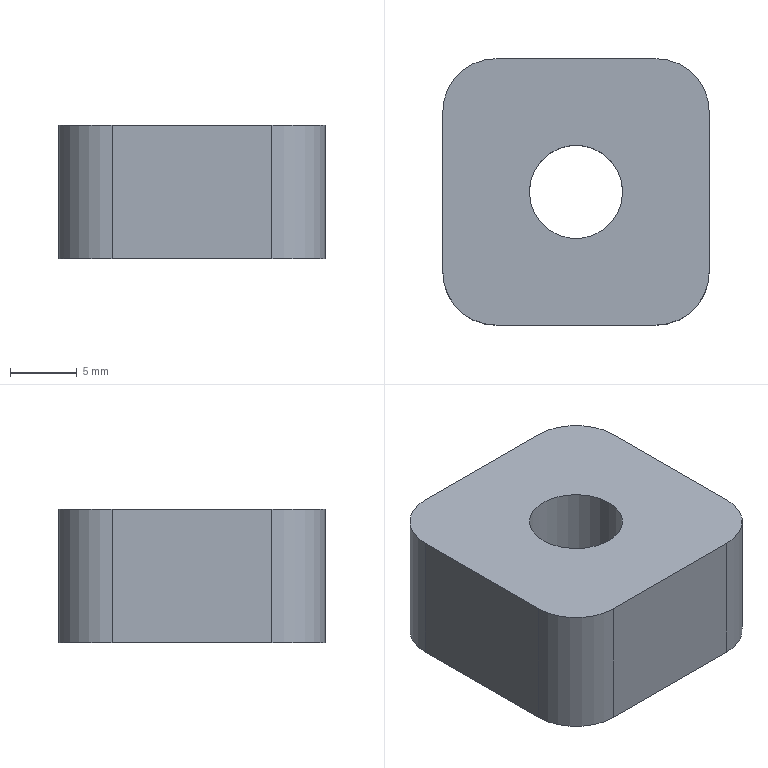Component | NX | FIX_BLOCK_3 | 1 solid | 11 faces | box 20 x 20 x 10 mm | volume 3478 mm3 | plane 6 | cylinder 5 | commonest cylinder face diameters 8 x4 7 x1
STEP:
#1=CARTESIAN_POINT('',(0.,0.,0.));
#2=DIRECTION('',(0.,0.,1.));
#3=DIRECTION('',(1.,0.,0.));
#4=AXIS2_PLACEMENT_3D('',#1,#2,#3);
#5=CARTESIAN_POINT('',(-10.,106.,0.));
#6=VERTEX_POINT('',#5);
#7=CARTESIAN_POINT('',(-10.,94.,0.));
#8=VERTEX_POINT('',#7);
#9=CARTESIAN_POINT('',(-10.,110.,0.));
#10=DIRECTION('',(0.,-1.,0.));
#11=VECTOR('',#10,1.);
#12=LINE('',#9,#11);
#13=CARTESIAN_POINT('',(-10.,110.,10.));
#14=DIRECTION('',(1.,0.,0.));
#15=DIRECTION('',(0.,0.,-1.));
#16=AXIS2_PLACEMENT_3D('',#13,#14,#15);
#17=PLANE('',#16);
#18=CARTESIAN_POINT('',(10.,0.));
#19=DIRECTION('',(0.,-1.));
#20=VECTOR('',#19,1.);
#21=LINE('',#18,#20);
#22=(GEOMETRIC_REPRESENTATION_CONTEXT(2)PARAMETRIC_REPRESENTATION_CONTEXT()REPRESENTATION_CONTEXT('',''));
#23=DEFINITIONAL_REPRESENTATION('',(#21),#22);
#24=PCURVE('',#17,#23);
#25=CARTESIAN_POINT('',(0.,100.,0.));
#26=DIRECTION('',(0.,0.,1.));
#27=DIRECTION('',(1.,0.,0.));
#28=AXIS2_PLACEMENT_3D('',#25,#26,#27);
#29=PLANE('',#28);
#30=CARTESIAN_POINT('',(-10.,10.));
#31=DIRECTION('',(0.,-1.));
#32=VECTOR('',#31,1.);
#33=LINE('',#30,#32);
#34=(GEOMETRIC_REPRESENTATION_CONTEXT(2)PARAMETRIC_REPRESENTATION_CONTEXT()REPRESENTATION_CONTEXT('',''));
#35=DEFINITIONAL_REPRESENTATION('',(#33),#34);
#36=PCURVE('',#29,#35);
#37=SURFACE_CURVE('',#12,(#24,#36),.PCURVE_S1.);
#38=EDGE_CURVE('',#6,#8,#37,.T.);
#39=ORIENTED_EDGE('',*,*,#38,.T.);
#40=CARTESIAN_POINT('',(-10.,94.,10.));
#41=VERTEX_POINT('',#40);
#42=CARTESIAN_POINT('',(-10.,94.,10.));
#43=DIRECTION('',(0.,0.,1.));
#44=VECTOR('',#43,1.);
#45=LINE('',#42,#44);
#46=CARTESIAN_POINT('',(0.,-16.));
#47=DIRECTION('',(-1.,0.));
#48=VECTOR('',#47,1.);
#49=LINE('',#46,#48);
#50=(GEOMETRIC_REPRESENTATION_CONTEXT(2)PARAMETRIC_REPRESENTATION_CONTEXT()REPRESENTATION_CONTEXT('',''));
#51=DEFINITIONAL_REPRESENTATION('',(#49),#50);
#52=PCURVE('',#17,#51);
#53=CARTESIAN_POINT('',(-6.,94.,10.));
#54=DIRECTION('',(0.,0.,-1.));
#55=DIRECTION('',(-1.,0.,0.));
#56=AXIS2_PLACEMENT_3D('',#53,#54,#55);
#57=CYLINDRICAL_SURFACE('',#56,4.);
#58=CARTESIAN_POINT('',(6.283,0.));
#59=DIRECTION('',(0.,-1.));
#60=VECTOR('',#59,1.);
#61=LINE('',#58,#60);
#62=(GEOMETRIC_REPRESENTATION_CONTEXT(2)PARAMETRIC_REPRESENTATION_CONTEXT()REPRESENTATION_CONTEXT('',''));
#63=DEFINITIONAL_REPRESENTATION('',(#61),#62);
#64=PCURVE('',#57,#63);
#65=SURFACE_CURVE('',#45,(#52,#64),.PCURVE_S1.);
#66=EDGE_CURVE('',#8,#41,#65,.T.);
#67=ORIENTED_EDGE('',*,*,#66,.T.);
#68=CARTESIAN_POINT('',(-10.,106.,10.));
#69=VERTEX_POINT('',#68);
#70=CARTESIAN_POINT('',(-10.,110.,10.));
#71=DIRECTION('',(0.,-1.,0.));
#72=VECTOR('',#71,1.);
#73=LINE('',#70,#72);
#74=CARTESIAN_POINT('',(0.,0.));
#75=DIRECTION('',(0.,-1.));
#76=VECTOR('',#75,1.);
#77=LINE('',#74,#76);
#78=(GEOMETRIC_REPRESENTATION_CONTEXT(2)PARAMETRIC_REPRESENTATION_CONTEXT()REPRESENTATION_CONTEXT('',''));
#79=DEFINITIONAL_REPRESENTATION('',(#77),#78);
#80=PCURVE('',#17,#79);
#81=CARTESIAN_POINT('',(0.,100.,10.));
#82=DIRECTION('',(0.,0.,1.));
#83=DIRECTION('',(1.,0.,0.));
#84=AXIS2_PLACEMENT_3D('',#81,#82,#83);
#85=PLANE('',#84);
#86=CARTESIAN_POINT('',(-10.,10.));
#87=DIRECTION('',(0.,-1.));
#88=VECTOR('',#87,1.);
#89=LINE('',#86,#88);
#90=(GEOMETRIC_REPRESENTATION_CONTEXT(2)PARAMETRIC_REPRESENTATION_CONTEXT()REPRESENTATION_CONTEXT('',''));
#91=DEFINITIONAL_REPRESENTATION('',(#89),#90);
#92=PCURVE('',#85,#91);
#93=SURFACE_CURVE('',#73,(#80,#92),.PCURVE_S1.);
#94=EDGE_CURVE('',#69,#41,#93,.T.);
#95=ORIENTED_EDGE('',*,*,#94,.F.);
#96=CARTESIAN_POINT('',(-10.,106.,10.));
#97=DIRECTION('',(0.,0.,-1.));
#98=VECTOR('',#97,1.);
#99=LINE('',#96,#98);
#100=CARTESIAN_POINT('',(0.,-4.));
#101=DIRECTION('',(1.,0.));
#102=VECTOR('',#101,1.);
#103=LINE('',#100,#102);
#104=(GEOMETRIC_REPRESENTATION_CONTEXT(2)PARAMETRIC_REPRESENTATION_CONTEXT()REPRESENTATION_CONTEXT('',''));
#105=DEFINITIONAL_REPRESENTATION('',(#103),#104);
#106=PCURVE('',#17,#105);
#107=CARTESIAN_POINT('',(-6.,106.,10.));
#108=DIRECTION('',(0.,0.,-1.));
#109=DIRECTION('',(-1.,0.,0.));
#110=AXIS2_PLACEMENT_3D('',#107,#108,#109);
#111=CYLINDRICAL_SURFACE('',#110,4.);
#112=CARTESIAN_POINT('',(0.,0.));
#113=DIRECTION('',(0.,1.));
#114=VECTOR('',#113,1.);
#115=LINE('',#112,#114);
#116=(GEOMETRIC_REPRESENTATION_CONTEXT(2)PARAMETRIC_REPRESENTATION_CONTEXT()REPRESENTATION_CONTEXT('',''));
#117=DEFINITIONAL_REPRESENTATION('',(#115),#116);
#118=PCURVE('',#111,#117);
#119=SURFACE_CURVE('',#99,(#106,#118),.PCURVE_S1.);
#120=EDGE_CURVE('',#69,#6,#119,.T.);
#121=ORIENTED_EDGE('',*,*,#120,.T.);
#122=EDGE_LOOP('',(#39,#67,#95,#121));
#123=FACE_BOUND('',#122,.T.);
#124=ADVANCED_FACE('',(#123),#17,.F.);
#125=CARTESIAN_POINT('',(-6.,90.,0.));
#126=VERTEX_POINT('',#125);
#127=CARTESIAN_POINT('',(6.,90.,0.));
#128=VERTEX_POINT('',#127);
#129=CARTESIAN_POINT('',(-10.,90.,0.));
#130=DIRECTION('',(1.,0.,0.));
#131=VECTOR('',#130,1.);
#132=LINE('',#129,#131);
#133=CARTESIAN_POINT('',(-10.,90.,10.));
#134=DIRECTION('',(0.,1.,0.));
#135=DIRECTION('',(0.,0.,1.));
#136=AXIS2_PLACEMENT_3D('',#133,#134,#135);
#137=PLANE('',#136);
#138=CARTESIAN_POINT('',(-10.,0.));
#139=DIRECTION('',(0.,1.));
#140=VECTOR('',#139,1.);
#141=LINE('',#138,#140);
#142=(GEOMETRIC_REPRESENTATION_CONTEXT(2)PARAMETRIC_REPRESENTATION_CONTEXT()REPRESENTATION_CONTEXT('',''));
#143=DEFINITIONAL_REPRESENTATION('',(#141),#142);
#144=PCURVE('',#137,#143);
#145=CARTESIAN_POINT('',(-10.,-10.));
#146=DIRECTION('',(1.,0.));
#147=VECTOR('',#146,1.);
#148=LINE('',#145,#147);
#149=(GEOMETRIC_REPRESENTATION_CONTEXT(2)PARAMETRIC_REPRESENTATION_CONTEXT()REPRESENTATION_CONTEXT('',''));
#150=DEFINITIONAL_REPRESENTATION('',(#148),#149);
#151=PCURVE('',#29,#150);
#152=SURFACE_CURVE('',#132,(#144,#151),.PCURVE_S1.);
#153=EDGE_CURVE('',#126,#128,#152,.T.);
#154=ORIENTED_EDGE('',*,*,#153,.T.);
#155=CARTESIAN_POINT('',(6.,90.,10.));
#156=VERTEX_POINT('',#155);
#157=CARTESIAN_POINT('',(6.,90.,10.));
#158=DIRECTION('',(0.,0.,1.));
#159=VECTOR('',#158,1.);
#160=LINE('',#157,#159);
#161=CARTESIAN_POINT('',(0.,16.));
#162=DIRECTION('',(1.,0.));
#163=VECTOR('',#162,1.);
#164=LINE('',#161,#163);
#165=(GEOMETRIC_REPRESENTATION_CONTEXT(2)PARAMETRIC_REPRESENTATION_CONTEXT()REPRESENTATION_CONTEXT('',''));
#166=DEFINITIONAL_REPRESENTATION('',(#164),#165);
#167=PCURVE('',#137,#166);
#168=CARTESIAN_POINT('',(6.,94.,10.));
#169=DIRECTION('',(0.,0.,-1.));
#170=DIRECTION('',(-1.,0.,0.));
#171=AXIS2_PLACEMENT_3D('',#168,#169,#170);
#172=CYLINDRICAL_SURFACE('',#171,4.);
#173=CARTESIAN_POINT('',(4.712,0.));
#174=DIRECTION('',(0.,-1.));
#175=VECTOR('',#174,1.);
#176=LINE('',#173,#175);
#177=(GEOMETRIC_REPRESENTATION_CONTEXT(2)PARAMETRIC_REPRESENTATION_CONTEXT()REPRESENTATION_CONTEXT('',''));
#178=DEFINITIONAL_REPRESENTATION('',(#176),#177);
#179=PCURVE('',#172,#178);
#180=SURFACE_CURVE('',#160,(#167,#179),.PCURVE_S1.);
#181=EDGE_CURVE('',#128,#156,#180,.T.);
#182=ORIENTED_EDGE('',*,*,#181,.T.);
#183=CARTESIAN_POINT('',(-6.,90.,10.));
#184=VERTEX_POINT('',#183);
#185=CARTESIAN_POINT('',(-10.,90.,10.));
#186=DIRECTION('',(1.,0.,0.));
#187=VECTOR('',#186,1.);
#188=LINE('',#185,#187);
#189=CARTESIAN_POINT('',(0.,0.));
#190=DIRECTION('',(0.,1.));
#191=VECTOR('',#190,1.);
#192=LINE('',#189,#191);
#193=(GEOMETRIC_REPRESENTATION_CONTEXT(2)PARAMETRIC_REPRESENTATION_CONTEXT()REPRESENTATION_CONTEXT('',''));
#194=DEFINITIONAL_REPRESENTATION('',(#192),#193);
#195=PCURVE('',#137,#194);
#196=CARTESIAN_POINT('',(-10.,-10.));
#197=DIRECTION('',(1.,0.));
#198=VECTOR('',#197,1.);
#199=LINE('',#196,#198);
#200=(GEOMETRIC_REPRESENTATION_CONTEXT(2)PARAMETRIC_REPRESENTATION_CONTEXT()REPRESENTATION_CONTEXT('',''));
#201=DEFINITIONAL_REPRESENTATION('',(#199),#200);
#202=PCURVE('',#85,#201);
#203=SURFACE_CURVE('',#188,(#195,#202),.PCURVE_S1.);
#204=EDGE_CURVE('',#184,#156,#203,.T.);
#205=ORIENTED_EDGE('',*,*,#204,.F.);
#206=CARTESIAN_POINT('',(-6.,90.,10.));
#207=DIRECTION('',(0.,0.,-1.));
#208=VECTOR('',#207,1.);
#209=LINE('',#206,#208);
#210=CARTESIAN_POINT('',(0.,4.));
#211=DIRECTION('',(-1.,0.));
#212=VECTOR('',#211,1.);
#213=LINE('',#210,#212);
#214=(GEOMETRIC_REPRESENTATION_CONTEXT(2)PARAMETRIC_REPRESENTATION_CONTEXT()REPRESENTATION_CONTEXT('',''));
#215=DEFINITIONAL_REPRESENTATION('',(#213),#214);
#216=PCURVE('',#137,#215);
#217=CARTESIAN_POINT('',(4.712,0.));
#218=DIRECTION('',(0.,1.));
#219=VECTOR('',#218,1.);
#220=LINE('',#217,#219);
#221=(GEOMETRIC_REPRESENTATION_CONTEXT(2)PARAMETRIC_REPRESENTATION_CONTEXT()REPRESENTATION_CONTEXT('',''));
#222=DEFINITIONAL_REPRESENTATION('',(#220),#221);
#223=PCURVE('',#57,#222);
#224=SURFACE_CURVE('',#209,(#216,#223),.PCURVE_S1.);
#225=EDGE_CURVE('',#184,#126,#224,.T.);
#226=ORIENTED_EDGE('',*,*,#225,.T.);
#227=EDGE_LOOP('',(#154,#182,#205,#226));
#228=FACE_BOUND('',#227,.T.);
#229=ADVANCED_FACE('',(#228),#137,.F.);
#230=CARTESIAN_POINT('',(10.,94.,10.));
#231=VERTEX_POINT('',#230);
#232=CARTESIAN_POINT('',(10.,106.,10.));
#233=VERTEX_POINT('',#232);
#234=CARTESIAN_POINT('',(10.,90.,10.));
#235=DIRECTION('',(0.,1.,0.));
#236=VECTOR('',#235,1.);
#237=LINE('',#234,#236);
#238=CARTESIAN_POINT('',(10.,90.,10.));
#239=DIRECTION('',(-1.,0.,0.));
#240=DIRECTION('',(0.,0.,1.));
#241=AXIS2_PLACEMENT_3D('',#238,#239,#240);
#242=PLANE('',#241);
#243=CARTESIAN_POINT('',(0.,0.));
#244=DIRECTION('',(0.,1.));
#245=VECTOR('',#244,1.);
#246=LINE('',#243,#245);
#247=(GEOMETRIC_REPRESENTATION_CONTEXT(2)PARAMETRIC_REPRESENTATION_CONTEXT()REPRESENTATION_CONTEXT('',''));
#248=DEFINITIONAL_REPRESENTATION('',(#246),#247);
#249=PCURVE('',#242,#248);
#250=CARTESIAN_POINT('',(10.,-10.));
#251=DIRECTION('',(0.,1.));
#252=VECTOR('',#251,1.);
#253=LINE('',#250,#252);
#254=(GEOMETRIC_REPRESENTATION_CONTEXT(2)PARAMETRIC_REPRESENTATION_CONTEXT()REPRESENTATION_CONTEXT('',''));
#255=DEFINITIONAL_REPRESENTATION('',(#253),#254);
#256=PCURVE('',#85,#255);
#257=SURFACE_CURVE('',#237,(#249,#256),.PCURVE_S1.);
#258=EDGE_CURVE('',#231,#233,#257,.T.);
#259=ORIENTED_EDGE('',*,*,#258,.F.);
#260=CARTESIAN_POINT('',(10.,94.,0.));
#261=VERTEX_POINT('',#260);
#262=CARTESIAN_POINT('',(10.,94.,10.));
#263=DIRECTION('',(0.,0.,-1.));
#264=VECTOR('',#263,1.);
#265=LINE('',#262,#264);
#266=CARTESIAN_POINT('',(0.,4.));
#267=DIRECTION('',(-1.,0.));
#268=VECTOR('',#267,1.);
#269=LINE('',#266,#268);
#270=(GEOMETRIC_REPRESENTATION_CONTEXT(2)PARAMETRIC_REPRESENTATION_CONTEXT()REPRESENTATION_CONTEXT('',''));
#271=DEFINITIONAL_REPRESENTATION('',(#269),#270);
#272=PCURVE('',#242,#271);
#273=CARTESIAN_POINT('',(3.142,0.));
#274=DIRECTION('',(0.,1.));
#275=VECTOR('',#274,1.);
#276=LINE('',#273,#275);
#277=(GEOMETRIC_REPRESENTATION_CONTEXT(2)PARAMETRIC_REPRESENTATION_CONTEXT()REPRESENTATION_CONTEXT('',''));
#278=DEFINITIONAL_REPRESENTATION('',(#276),#277);
#279=PCURVE('',#172,#278);
#280=SURFACE_CURVE('',#265,(#272,#279),.PCURVE_S1.);
#281=EDGE_CURVE('',#231,#261,#280,.T.);
#282=ORIENTED_EDGE('',*,*,#281,.T.);
#283=CARTESIAN_POINT('',(10.,106.,0.));
#284=VERTEX_POINT('',#283);
#285=CARTESIAN_POINT('',(10.,90.,0.));
#286=DIRECTION('',(0.,1.,0.));
#287=VECTOR('',#286,1.);
#288=LINE('',#285,#287);
#289=CARTESIAN_POINT('',(-10.,0.));
#290=DIRECTION('',(0.,1.));
#291=VECTOR('',#290,1.);
#292=LINE('',#289,#291);
#293=(GEOMETRIC_REPRESENTATION_CONTEXT(2)PARAMETRIC_REPRESENTATION_CONTEXT()REPRESENTATION_CONTEXT('',''));
#294=DEFINITIONAL_REPRESENTATION('',(#292),#293);
#295=PCURVE('',#242,#294);
#296=CARTESIAN_POINT('',(10.,-10.));
#297=DIRECTION('',(0.,1.));
#298=VECTOR('',#297,1.);
#299=LINE('',#296,#298);
#300=(GEOMETRIC_REPRESENTATION_CONTEXT(2)PARAMETRIC_REPRESENTATION_CONTEXT()REPRESENTATION_CONTEXT('',''));
#301=DEFINITIONAL_REPRESENTATION('',(#299),#300);
#302=PCURVE('',#29,#301);
#303=SURFACE_CURVE('',#288,(#295,#302),.PCURVE_S1.);
#304=EDGE_CURVE('',#261,#284,#303,.T.);
#305=ORIENTED_EDGE('',*,*,#304,.T.);
#306=CARTESIAN_POINT('',(10.,106.,10.));
#307=DIRECTION('',(0.,0.,1.));
#308=VECTOR('',#307,1.);
#309=LINE('',#306,#308);
#310=CARTESIAN_POINT('',(0.,16.));
#311=DIRECTION('',(1.,0.));
#312=VECTOR('',#311,1.);
#313=LINE('',#310,#312);
#314=(GEOMETRIC_REPRESENTATION_CONTEXT(2)PARAMETRIC_REPRESENTATION_CONTEXT()REPRESENTATION_CONTEXT('',''));
#315=DEFINITIONAL_REPRESENTATION('',(#313),#314);
#316=PCURVE('',#242,#315);
#317=CARTESIAN_POINT('',(6.,106.,10.));
#318=DIRECTION('',(0.,0.,-1.));
#319=DIRECTION('',(-1.,0.,0.));
#320=AXIS2_PLACEMENT_3D('',#317,#318,#319);
#321=CYLINDRICAL_SURFACE('',#320,4.);
#322=CARTESIAN_POINT('',(3.142,0.));
#323=DIRECTION('',(0.,-1.));
#324=VECTOR('',#323,1.);
#325=LINE('',#322,#324);
#326=(GEOMETRIC_REPRESENTATION_CONTEXT(2)PARAMETRIC_REPRESENTATION_CONTEXT()REPRESENTATION_CONTEXT('',''));
#327=DEFINITIONAL_REPRESENTATION('',(#325),#326);
#328=PCURVE('',#321,#327);
#329=SURFACE_CURVE('',#309,(#316,#328),.PCURVE_S1.);
#330=EDGE_CURVE('',#284,#233,#329,.T.);
#331=ORIENTED_EDGE('',*,*,#330,.T.);
#332=EDGE_LOOP('',(#259,#282,#305,#331));
#333=FACE_BOUND('',#332,.T.);
#334=ADVANCED_FACE('',(#333),#242,.F.);
#335=CARTESIAN_POINT('',(6.,110.,10.));
#336=VERTEX_POINT('',#335);
#337=CARTESIAN_POINT('',(-6.,110.,10.));
#338=VERTEX_POINT('',#337);
#339=CARTESIAN_POINT('',(10.,110.,10.));
#340=DIRECTION('',(-1.,0.,0.));
#341=VECTOR('',#340,1.);
#342=LINE('',#339,#341);
#343=CARTESIAN_POINT('',(10.,110.,10.));
#344=DIRECTION('',(0.,-1.,0.));
#345=DIRECTION('',(0.,0.,-1.));
#346=AXIS2_PLACEMENT_3D('',#343,#344,#345);
#347=PLANE('',#346);
#348=CARTESIAN_POINT('',(0.,0.));
#349=DIRECTION('',(0.,-1.));
#350=VECTOR('',#349,1.);
#351=LINE('',#348,#350);
#352=(GEOMETRIC_REPRESENTATION_CONTEXT(2)PARAMETRIC_REPRESENTATION_CONTEXT()REPRESENTATION_CONTEXT('',''));
#353=DEFINITIONAL_REPRESENTATION('',(#351),#352);
#354=PCURVE('',#347,#353);
#355=CARTESIAN_POINT('',(10.,10.));
#356=DIRECTION('',(-1.,0.));
#357=VECTOR('',#356,1.);
#358=LINE('',#355,#357);
#359=(GEOMETRIC_REPRESENTATION_CONTEXT(2)PARAMETRIC_REPRESENTATION_CONTEXT()REPRESENTATION_CONTEXT('',''));
#360=DEFINITIONAL_REPRESENTATION('',(#358),#359);
#361=PCURVE('',#85,#360);
#362=SURFACE_CURVE('',#342,(#354,#361),.PCURVE_S1.);
#363=EDGE_CURVE('',#336,#338,#362,.T.);
#364=ORIENTED_EDGE('',*,*,#363,.F.);
#365=CARTESIAN_POINT('',(6.,110.,0.));
#366=VERTEX_POINT('',#365);
#367=CARTESIAN_POINT('',(6.,110.,10.));
#368=DIRECTION('',(0.,0.,-1.));
#369=VECTOR('',#368,1.);
#370=LINE('',#367,#369);
#371=CARTESIAN_POINT('',(0.,-4.));
#372=DIRECTION('',(1.,0.));
#373=VECTOR('',#372,1.);
#374=LINE('',#371,#373);
#375=(GEOMETRIC_REPRESENTATION_CONTEXT(2)PARAMETRIC_REPRESENTATION_CONTEXT()REPRESENTATION_CONTEXT('',''));
#376=DEFINITIONAL_REPRESENTATION('',(#374),#375);
#377=PCURVE('',#347,#376);
#378=CARTESIAN_POINT('',(1.571,0.));
#379=DIRECTION('',(0.,1.));
#380=VECTOR('',#379,1.);
#381=LINE('',#378,#380);
#382=(GEOMETRIC_REPRESENTATION_CONTEXT(2)PARAMETRIC_REPRESENTATION_CONTEXT()REPRESENTATION_CONTEXT('',''));
#383=DEFINITIONAL_REPRESENTATION('',(#381),#382);
#384=PCURVE('',#321,#383);
#385=SURFACE_CURVE('',#370,(#377,#384),.PCURVE_S1.);
#386=EDGE_CURVE('',#336,#366,#385,.T.);
#387=ORIENTED_EDGE('',*,*,#386,.T.);
#388=CARTESIAN_POINT('',(-6.,110.,0.));
#389=VERTEX_POINT('',#388);
#390=CARTESIAN_POINT('',(10.,110.,0.));
#391=DIRECTION('',(-1.,0.,0.));
#392=VECTOR('',#391,1.);
#393=LINE('',#390,#392);
#394=CARTESIAN_POINT('',(10.,0.));
#395=DIRECTION('',(0.,-1.));
#396=VECTOR('',#395,1.);
#397=LINE('',#394,#396);
#398=(GEOMETRIC_REPRESENTATION_CONTEXT(2)PARAMETRIC_REPRESENTATION_CONTEXT()REPRESENTATION_CONTEXT('',''));
#399=DEFINITIONAL_REPRESENTATION('',(#397),#398);
#400=PCURVE('',#347,#399);
#401=CARTESIAN_POINT('',(10.,10.));
#402=DIRECTION('',(-1.,0.));
#403=VECTOR('',#402,1.);
#404=LINE('',#401,#403);
#405=(GEOMETRIC_REPRESENTATION_CONTEXT(2)PARAMETRIC_REPRESENTATION_CONTEXT()REPRESENTATION_CONTEXT('',''));
#406=DEFINITIONAL_REPRESENTATION('',(#404),#405);
#407=PCURVE('',#29,#406);
#408=SURFACE_CURVE('',#393,(#400,#407),.PCURVE_S1.);
#409=EDGE_CURVE('',#366,#389,#408,.T.);
#410=ORIENTED_EDGE('',*,*,#409,.T.);
#411=CARTESIAN_POINT('',(-6.,110.,10.));
#412=DIRECTION('',(0.,0.,1.));
#413=VECTOR('',#412,1.);
#414=LINE('',#411,#413);
#415=CARTESIAN_POINT('',(0.,-16.));
#416=DIRECTION('',(-1.,0.));
#417=VECTOR('',#416,1.);
#418=LINE('',#415,#417);
#419=(GEOMETRIC_REPRESENTATION_CONTEXT(2)PARAMETRIC_REPRESENTATION_CONTEXT()REPRESENTATION_CONTEXT('',''));
#420=DEFINITIONAL_REPRESENTATION('',(#418),#419);
#421=PCURVE('',#347,#420);
#422=CARTESIAN_POINT('',(1.571,0.));
#423=DIRECTION('',(0.,-1.));
#424=VECTOR('',#423,1.);
#425=LINE('',#422,#424);
#426=(GEOMETRIC_REPRESENTATION_CONTEXT(2)PARAMETRIC_REPRESENTATION_CONTEXT()REPRESENTATION_CONTEXT('',''));
#427=DEFINITIONAL_REPRESENTATION('',(#425),#426);
#428=PCURVE('',#111,#427);
#429=SURFACE_CURVE('',#414,(#421,#428),.PCURVE_S1.);
#430=EDGE_CURVE('',#389,#338,#429,.T.);
#431=ORIENTED_EDGE('',*,*,#430,.T.);
#432=EDGE_LOOP('',(#364,#387,#410,#431));
#433=FACE_BOUND('',#432,.T.);
#434=ADVANCED_FACE('',(#433),#347,.F.);
#435=CARTESIAN_POINT('',(3.5,100.,10.));
#436=VERTEX_POINT('',#435);
#437=CARTESIAN_POINT('',(0.,100.,10.));
#438=DIRECTION('',(0.,0.,1.));
#439=DIRECTION('',(1.,0.,0.));
#440=AXIS2_PLACEMENT_3D('',#437,#438,#439);
#441=CIRCLE('',#440,3.5);
#442=CARTESIAN_POINT('',(0.,100.,10.));
#443=DIRECTION('',(0.,0.,-1.));
#444=DIRECTION('',(-1.,0.,0.));
#445=AXIS2_PLACEMENT_3D('',#442,#443,#444);
#446=CYLINDRICAL_SURFACE('',#445,3.5);
#447=CARTESIAN_POINT('',(9.425,0.));
#448=DIRECTION('',(-1.,0.));
#449=VECTOR('',#448,1.);
#450=LINE('',#447,#449);
#451=(GEOMETRIC_REPRESENTATION_CONTEXT(2)PARAMETRIC_REPRESENTATION_CONTEXT()REPRESENTATION_CONTEXT('',''));
#452=DEFINITIONAL_REPRESENTATION('',(#450),#451);
#453=PCURVE('',#446,#452);
#454=CARTESIAN_POINT('',(0.,0.));
#455=DIRECTION('',(1.,0.));
#456=AXIS2_PLACEMENT_2D('',#454,#455);
#457=CIRCLE('',#456,3.5);
#458=(GEOMETRIC_REPRESENTATION_CONTEXT(2)PARAMETRIC_REPRESENTATION_CONTEXT()REPRESENTATION_CONTEXT('',''));
#459=DEFINITIONAL_REPRESENTATION('',(#457),#458);
#460=PCURVE('',#85,#459);
#461=SURFACE_CURVE('',#441,(#453,#460),.PCURVE_S1.);
#462=EDGE_CURVE('',#436,#436,#461,.T.);
#463=ORIENTED_EDGE('',*,*,#462,.F.);
#464=CARTESIAN_POINT('',(3.5,100.,0.));
#465=VERTEX_POINT('',#464);
#466=CARTESIAN_POINT('',(3.5,100.,10.));
#467=CARTESIAN_POINT('',(3.5,100.,0.));
#468=B_SPLINE_CURVE_WITH_KNOTS('',1,(#466,#467),.UNSPECIFIED.,.F.,.F.,(2,2),(0.,10.),.PIECEWISE_BEZIER_KNOTS.);
#469=CARTESIAN_POINT('',(9.425,0.));
#470=DIRECTION('',(0.,1.));
#471=VECTOR('',#470,1.);
#472=LINE('',#469,#471);
#473=(GEOMETRIC_REPRESENTATION_CONTEXT(2)PARAMETRIC_REPRESENTATION_CONTEXT()REPRESENTATION_CONTEXT('',''));
#474=DEFINITIONAL_REPRESENTATION('',(#472),#473);
#475=PCURVE('',#446,#474);
#476=CARTESIAN_POINT('',(3.142,0.));
#477=DIRECTION('',(0.,1.));
#478=VECTOR('',#477,1.);
#479=LINE('',#476,#478);
#480=(GEOMETRIC_REPRESENTATION_CONTEXT(2)PARAMETRIC_REPRESENTATION_CONTEXT()REPRESENTATION_CONTEXT('',''));
#481=DEFINITIONAL_REPRESENTATION('',(#479),#480);
#482=PCURVE('',#446,#481);
#483=SEAM_CURVE('',#468,(#475,#482),.PCURVE_S1.);
#484=EDGE_CURVE('',#436,#465,#483,.T.);
#485=ORIENTED_EDGE('',*,*,#484,.T.);
#486=CARTESIAN_POINT('',(0.,100.,0.));
#487=DIRECTION('',(0.,0.,1.));
#488=DIRECTION('',(1.,0.,0.));
#489=AXIS2_PLACEMENT_3D('',#486,#487,#488);
#490=CIRCLE('',#489,3.5);
#491=CARTESIAN_POINT('',(9.425,10.));
#492=DIRECTION('',(-1.,0.));
#493=VECTOR('',#492,1.);
#494=LINE('',#491,#493);
#495=(GEOMETRIC_REPRESENTATION_CONTEXT(2)PARAMETRIC_REPRESENTATION_CONTEXT()REPRESENTATION_CONTEXT('',''));
#496=DEFINITIONAL_REPRESENTATION('',(#494),#495);
#497=PCURVE('',#446,#496);
#498=CARTESIAN_POINT('',(0.,0.));
#499=DIRECTION('',(1.,0.));
#500=AXIS2_PLACEMENT_2D('',#498,#499);
#501=CIRCLE('',#500,3.5);
#502=(GEOMETRIC_REPRESENTATION_CONTEXT(2)PARAMETRIC_REPRESENTATION_CONTEXT()REPRESENTATION_CONTEXT('',''));
#503=DEFINITIONAL_REPRESENTATION('',(#501),#502);
#504=PCURVE('',#29,#503);
#505=SURFACE_CURVE('',#490,(#497,#504),.PCURVE_S1.);
#506=EDGE_CURVE('',#465,#465,#505,.T.);
#507=ORIENTED_EDGE('',*,*,#506,.T.);
#508=ORIENTED_EDGE('',*,*,#484,.F.);
#509=EDGE_LOOP('',(#463,#485,#507,#508));
#510=FACE_BOUND('',#509,.F.);
#511=ADVANCED_FACE('',(#510),#446,.F.);
#512=ORIENTED_EDGE('',*,*,#204,.T.);
#513=CARTESIAN_POINT('',(6.,94.,10.));
#514=DIRECTION('',(0.,0.,1.));
#515=DIRECTION('',(1.,0.,0.));
#516=AXIS2_PLACEMENT_3D('',#513,#514,#515);
#517=CIRCLE('',#516,4.);
#518=CARTESIAN_POINT('',(6.,-6.));
#519=DIRECTION('',(1.,0.));
#520=AXIS2_PLACEMENT_2D('',#518,#519);
#521=CIRCLE('',#520,4.);
#522=(GEOMETRIC_REPRESENTATION_CONTEXT(2)PARAMETRIC_REPRESENTATION_CONTEXT()REPRESENTATION_CONTEXT('',''));
#523=DEFINITIONAL_REPRESENTATION('',(#521),#522);
#524=PCURVE('',#85,#523);
#525=CARTESIAN_POINT('',(9.425,0.));
#526=DIRECTION('',(-1.,0.));
#527=VECTOR('',#526,1.);
#528=LINE('',#525,#527);
#529=(GEOMETRIC_REPRESENTATION_CONTEXT(2)PARAMETRIC_REPRESENTATION_CONTEXT()REPRESENTATION_CONTEXT('',''));
#530=DEFINITIONAL_REPRESENTATION('',(#528),#529);
#531=PCURVE('',#172,#530);
#532=SURFACE_CURVE('',#517,(#524,#531),.PCURVE_S1.);
#533=EDGE_CURVE('',#156,#231,#532,.T.);
#534=ORIENTED_EDGE('',*,*,#533,.T.);
#535=ORIENTED_EDGE('',*,*,#258,.T.);
#536=CARTESIAN_POINT('',(6.,106.,10.));
#537=DIRECTION('',(0.,0.,1.));
#538=DIRECTION('',(1.,0.,0.));
#539=AXIS2_PLACEMENT_3D('',#536,#537,#538);
#540=CIRCLE('',#539,4.);
#541=CARTESIAN_POINT('',(6.,6.));
#542=DIRECTION('',(1.,0.));
#543=AXIS2_PLACEMENT_2D('',#541,#542);
#544=CIRCLE('',#543,4.);
#545=(GEOMETRIC_REPRESENTATION_CONTEXT(2)PARAMETRIC_REPRESENTATION_CONTEXT()REPRESENTATION_CONTEXT('',''));
#546=DEFINITIONAL_REPRESENTATION('',(#544),#545);
#547=PCURVE('',#85,#546);
#548=CARTESIAN_POINT('',(3.142,0.));
#549=DIRECTION('',(-1.,0.));
#550=VECTOR('',#549,1.);
#551=LINE('',#548,#550);
#552=(GEOMETRIC_REPRESENTATION_CONTEXT(2)PARAMETRIC_REPRESENTATION_CONTEXT()REPRESENTATION_CONTEXT('',''));
#553=DEFINITIONAL_REPRESENTATION('',(#551),#552);
#554=PCURVE('',#321,#553);
#555=SURFACE_CURVE('',#540,(#547,#554),.PCURVE_S1.);
#556=EDGE_CURVE('',#233,#336,#555,.T.);
#557=ORIENTED_EDGE('',*,*,#556,.T.);
#558=ORIENTED_EDGE('',*,*,#363,.T.);
#559=CARTESIAN_POINT('',(-6.,106.,10.));
#560=DIRECTION('',(0.,0.,1.));
#561=DIRECTION('',(1.,0.,0.));
#562=AXIS2_PLACEMENT_3D('',#559,#560,#561);
#563=CIRCLE('',#562,4.);
#564=CARTESIAN_POINT('',(-6.,6.));
#565=DIRECTION('',(1.,0.));
#566=AXIS2_PLACEMENT_2D('',#564,#565);
#567=CIRCLE('',#566,4.);
#568=(GEOMETRIC_REPRESENTATION_CONTEXT(2)PARAMETRIC_REPRESENTATION_CONTEXT()REPRESENTATION_CONTEXT('',''));
#569=DEFINITIONAL_REPRESENTATION('',(#567),#568);
#570=PCURVE('',#85,#569);
#571=CARTESIAN_POINT('',(3.142,0.));
#572=DIRECTION('',(-1.,0.));
#573=VECTOR('',#572,1.);
#574=LINE('',#571,#573);
#575=(GEOMETRIC_REPRESENTATION_CONTEXT(2)PARAMETRIC_REPRESENTATION_CONTEXT()REPRESENTATION_CONTEXT('',''));
#576=DEFINITIONAL_REPRESENTATION('',(#574),#575);
#577=PCURVE('',#111,#576);
#578=SURFACE_CURVE('',#563,(#570,#577),.PCURVE_S1.);
#579=EDGE_CURVE('',#338,#69,#578,.T.);
#580=ORIENTED_EDGE('',*,*,#579,.T.);
#581=ORIENTED_EDGE('',*,*,#94,.T.);
#582=CARTESIAN_POINT('',(-6.,94.,10.));
#583=DIRECTION('',(0.,0.,1.));
#584=DIRECTION('',(1.,0.,0.));
#585=AXIS2_PLACEMENT_3D('',#582,#583,#584);
#586=CIRCLE('',#585,4.);
#587=CARTESIAN_POINT('',(-6.,-6.));
#588=DIRECTION('',(1.,0.));
#589=AXIS2_PLACEMENT_2D('',#587,#588);
#590=CIRCLE('',#589,4.);
#591=(GEOMETRIC_REPRESENTATION_CONTEXT(2)PARAMETRIC_REPRESENTATION_CONTEXT()REPRESENTATION_CONTEXT('',''));
#592=DEFINITIONAL_REPRESENTATION('',(#590),#591);
#593=PCURVE('',#85,#592);
#594=CARTESIAN_POINT('',(9.425,0.));
#595=DIRECTION('',(-1.,0.));
#596=VECTOR('',#595,1.);
#597=LINE('',#594,#596);
#598=(GEOMETRIC_REPRESENTATION_CONTEXT(2)PARAMETRIC_REPRESENTATION_CONTEXT()REPRESENTATION_CONTEXT('',''));
#599=DEFINITIONAL_REPRESENTATION('',(#597),#598);
#600=PCURVE('',#57,#599);
#601=SURFACE_CURVE('',#586,(#593,#600),.PCURVE_S1.);
#602=EDGE_CURVE('',#41,#184,#601,.T.);
#603=ORIENTED_EDGE('',*,*,#602,.T.);
#604=EDGE_LOOP('',(#512,#534,#535,#557,#558,#580,#581,#603));
#605=FACE_BOUND('',#604,.T.);
#606=ORIENTED_EDGE('',*,*,#462,.F.);
#607=EDGE_LOOP('',(#606));
#608=FACE_BOUND('',#607,.T.);
#609=ADVANCED_FACE('',(#605,#608),#85,.T.);
#610=ORIENTED_EDGE('',*,*,#304,.F.);
#611=CARTESIAN_POINT('',(6.,94.,0.));
#612=DIRECTION('',(0.,0.,-1.));
#613=DIRECTION('',(1.,0.,0.));
#614=AXIS2_PLACEMENT_3D('',#611,#612,#613);
#615=CIRCLE('',#614,4.);
#616=CARTESIAN_POINT('',(10.,-6.));
#617=CARTESIAN_POINT('',(10.,-12.928));
#618=CARTESIAN_POINT('',(4.,-9.464));
#619=CARTESIAN_POINT('',(-2.,-6.));
#620=CARTESIAN_POINT('',(4.,-2.536));
#621=CARTESIAN_POINT('',(10.,0.9282));
#622=CARTESIAN_POINT('',(10.,-6.));
#623=(BOUNDED_CURVE()B_SPLINE_CURVE(2,(#616,#617,#618,#619,#620,#621,#622),.UNSPECIFIED.,.T.,.F.)B_SPLINE_CURVE_WITH_KNOTS((1,2,2,2,2,1),(-2.094,0.,2.094,4.189,6.283,8.378),.UNSPECIFIED.)CURVE()GEOMETRIC_REPRESENTATION_ITEM()RATIONAL_B_SPLINE_CURVE((1.,0.5,1.,0.5,1.,0.5,1.))REPRESENTATION_ITEM(''));
#624=(GEOMETRIC_REPRESENTATION_CONTEXT(2)PARAMETRIC_REPRESENTATION_CONTEXT()REPRESENTATION_CONTEXT('',''));
#625=DEFINITIONAL_REPRESENTATION('',(#623),#624);
#626=PCURVE('',#29,#625);
#627=CARTESIAN_POINT('',(3.142,10.));
#628=DIRECTION('',(1.,0.));
#629=VECTOR('',#628,1.);
#630=LINE('',#627,#629);
#631=(GEOMETRIC_REPRESENTATION_CONTEXT(2)PARAMETRIC_REPRESENTATION_CONTEXT()REPRESENTATION_CONTEXT('',''));
#632=DEFINITIONAL_REPRESENTATION('',(#630),#631);
#633=PCURVE('',#172,#632);
#634=SURFACE_CURVE('',#615,(#626,#633),.PCURVE_S1.);
#635=EDGE_CURVE('',#261,#128,#634,.T.);
#636=ORIENTED_EDGE('',*,*,#635,.T.);
#637=ORIENTED_EDGE('',*,*,#153,.F.);
#638=CARTESIAN_POINT('',(-6.,94.,0.));
#639=DIRECTION('',(0.,0.,-1.));
#640=DIRECTION('',(1.,0.,0.));
#641=AXIS2_PLACEMENT_3D('',#638,#639,#640);
#642=CIRCLE('',#641,4.);
#643=CARTESIAN_POINT('',(-2.,-6.));
#644=CARTESIAN_POINT('',(-2.,-12.928));
#645=CARTESIAN_POINT('',(-8.,-9.464));
#646=CARTESIAN_POINT('',(-14.,-6.));
#647=CARTESIAN_POINT('',(-8.,-2.536));
#648=CARTESIAN_POINT('',(-2.,0.9282));
#649=CARTESIAN_POINT('',(-2.,-6.));
#650=(BOUNDED_CURVE()B_SPLINE_CURVE(2,(#643,#644,#645,#646,#647,#648,#649),.UNSPECIFIED.,.T.,.F.)B_SPLINE_CURVE_WITH_KNOTS((1,2,2,2,2,1),(-2.094,0.,2.094,4.189,6.283,8.378),.UNSPECIFIED.)CURVE()GEOMETRIC_REPRESENTATION_ITEM()RATIONAL_B_SPLINE_CURVE((1.,0.5,1.,0.5,1.,0.5,1.))REPRESENTATION_ITEM(''));
#651=(GEOMETRIC_REPRESENTATION_CONTEXT(2)PARAMETRIC_REPRESENTATION_CONTEXT()REPRESENTATION_CONTEXT('',''));
#652=DEFINITIONAL_REPRESENTATION('',(#650),#651);
#653=PCURVE('',#29,#652);
#654=CARTESIAN_POINT('',(3.142,10.));
#655=DIRECTION('',(1.,0.));
#656=VECTOR('',#655,1.);
#657=LINE('',#654,#656);
#658=(GEOMETRIC_REPRESENTATION_CONTEXT(2)PARAMETRIC_REPRESENTATION_CONTEXT()REPRESENTATION_CONTEXT('',''));
#659=DEFINITIONAL_REPRESENTATION('',(#657),#658);
#660=PCURVE('',#57,#659);
#661=SURFACE_CURVE('',#642,(#653,#660),.PCURVE_S1.);
#662=EDGE_CURVE('',#126,#8,#661,.T.);
#663=ORIENTED_EDGE('',*,*,#662,.T.);
#664=ORIENTED_EDGE('',*,*,#38,.F.);
#665=CARTESIAN_POINT('',(-6.,106.,0.));
#666=DIRECTION('',(0.,0.,-1.));
#667=DIRECTION('',(1.,0.,0.));
#668=AXIS2_PLACEMENT_3D('',#665,#666,#667);
#669=CIRCLE('',#668,4.);
#670=CARTESIAN_POINT('',(-2.,6.));
#671=CARTESIAN_POINT('',(-2.,-0.9282));
#672=CARTESIAN_POINT('',(-8.,2.536));
#673=CARTESIAN_POINT('',(-14.,6.));
#674=CARTESIAN_POINT('',(-8.,9.464));
#675=CARTESIAN_POINT('',(-2.,12.928));
#676=CARTESIAN_POINT('',(-2.,6.));
#677=(BOUNDED_CURVE()B_SPLINE_CURVE(2,(#670,#671,#672,#673,#674,#675,#676),.UNSPECIFIED.,.T.,.F.)B_SPLINE_CURVE_WITH_KNOTS((1,2,2,2,2,1),(-2.094,0.,2.094,4.189,6.283,8.378),.UNSPECIFIED.)CURVE()GEOMETRIC_REPRESENTATION_ITEM()RATIONAL_B_SPLINE_CURVE((1.,0.5,1.,0.5,1.,0.5,1.))REPRESENTATION_ITEM(''));
#678=(GEOMETRIC_REPRESENTATION_CONTEXT(2)PARAMETRIC_REPRESENTATION_CONTEXT()REPRESENTATION_CONTEXT('',''));
#679=DEFINITIONAL_REPRESENTATION('',(#677),#678);
#680=PCURVE('',#29,#679);
#681=CARTESIAN_POINT('',(-3.142,10.));
#682=DIRECTION('',(1.,0.));
#683=VECTOR('',#682,1.);
#684=LINE('',#681,#683);
#685=(GEOMETRIC_REPRESENTATION_CONTEXT(2)PARAMETRIC_REPRESENTATION_CONTEXT()REPRESENTATION_CONTEXT('',''));
#686=DEFINITIONAL_REPRESENTATION('',(#684),#685);
#687=PCURVE('',#111,#686);
#688=SURFACE_CURVE('',#669,(#680,#687),.PCURVE_S1.);
#689=EDGE_CURVE('',#6,#389,#688,.T.);
#690=ORIENTED_EDGE('',*,*,#689,.T.);
#691=ORIENTED_EDGE('',*,*,#409,.F.);
#692=CARTESIAN_POINT('',(6.,106.,0.));
#693=DIRECTION('',(0.,0.,-1.));
#694=DIRECTION('',(1.,0.,0.));
#695=AXIS2_PLACEMENT_3D('',#692,#693,#694);
#696=CIRCLE('',#695,4.);
#697=CARTESIAN_POINT('',(10.,6.));
#698=CARTESIAN_POINT('',(10.,-0.9282));
#699=CARTESIAN_POINT('',(4.,2.536));
#700=CARTESIAN_POINT('',(-2.,6.));
#701=CARTESIAN_POINT('',(4.,9.464));
#702=CARTESIAN_POINT('',(10.,12.928));
#703=CARTESIAN_POINT('',(10.,6.));
#704=(BOUNDED_CURVE()B_SPLINE_CURVE(2,(#697,#698,#699,#700,#701,#702,#703),.UNSPECIFIED.,.T.,.F.)B_SPLINE_CURVE_WITH_KNOTS((1,2,2,2,2,1),(-2.094,0.,2.094,4.189,6.283,8.378),.UNSPECIFIED.)CURVE()GEOMETRIC_REPRESENTATION_ITEM()RATIONAL_B_SPLINE_CURVE((1.,0.5,1.,0.5,1.,0.5,1.))REPRESENTATION_ITEM(''));
#705=(GEOMETRIC_REPRESENTATION_CONTEXT(2)PARAMETRIC_REPRESENTATION_CONTEXT()REPRESENTATION_CONTEXT('',''));
#706=DEFINITIONAL_REPRESENTATION('',(#704),#705);
#707=PCURVE('',#29,#706);
#708=CARTESIAN_POINT('',(-3.142,10.));
#709=DIRECTION('',(1.,0.));
#710=VECTOR('',#709,1.);
#711=LINE('',#708,#710);
#712=(GEOMETRIC_REPRESENTATION_CONTEXT(2)PARAMETRIC_REPRESENTATION_CONTEXT()REPRESENTATION_CONTEXT('',''));
#713=DEFINITIONAL_REPRESENTATION('',(#711),#712);
#714=PCURVE('',#321,#713);
#715=SURFACE_CURVE('',#696,(#707,#714),.PCURVE_S1.);
#716=EDGE_CURVE('',#366,#284,#715,.T.);
#717=ORIENTED_EDGE('',*,*,#716,.T.);
#718=EDGE_LOOP('',(#610,#636,#637,#663,#664,#690,#691,#717));
#719=FACE_BOUND('',#718,.T.);
#720=ORIENTED_EDGE('',*,*,#506,.T.);
#721=EDGE_LOOP('',(#720));
#722=FACE_BOUND('',#721,.T.);
#723=ADVANCED_FACE('',(#719,#722),#29,.F.);
#724=ORIENTED_EDGE('',*,*,#533,.F.);
#725=ORIENTED_EDGE('',*,*,#181,.F.);
#726=ORIENTED_EDGE('',*,*,#635,.F.);
#727=ORIENTED_EDGE('',*,*,#281,.F.);
#728=EDGE_LOOP('',(#724,#725,#726,#727));
#729=FACE_BOUND('',#728,.T.);
#730=ADVANCED_FACE('',(#729),#172,.T.);
#731=ORIENTED_EDGE('',*,*,#602,.F.);
#732=ORIENTED_EDGE('',*,*,#66,.F.);
#733=ORIENTED_EDGE('',*,*,#662,.F.);
#734=ORIENTED_EDGE('',*,*,#225,.F.);
#735=EDGE_LOOP('',(#731,#732,#733,#734));
#736=FACE_BOUND('',#735,.T.);
#737=ADVANCED_FACE('',(#736),#57,.T.);
#738=ORIENTED_EDGE('',*,*,#556,.F.);
#739=ORIENTED_EDGE('',*,*,#330,.F.);
#740=ORIENTED_EDGE('',*,*,#716,.F.);
#741=ORIENTED_EDGE('',*,*,#386,.F.);
#742=EDGE_LOOP('',(#738,#739,#740,#741));
#743=FACE_BOUND('',#742,.T.);
#744=ADVANCED_FACE('',(#743),#321,.T.);
#745=ORIENTED_EDGE('',*,*,#579,.F.);
#746=ORIENTED_EDGE('',*,*,#430,.F.);
#747=ORIENTED_EDGE('',*,*,#689,.F.);
#748=ORIENTED_EDGE('',*,*,#120,.F.);
#749=EDGE_LOOP('',(#745,#746,#747,#748));
#750=FACE_BOUND('',#749,.T.);
#751=ADVANCED_FACE('',(#750),#111,.T.);
#752=CLOSED_SHELL('',(#124,#229,#334,#434,#511,#609,#723,#730,#737,#744,#751));
#753=MANIFOLD_SOLID_BREP('',#752);
#754=(LENGTH_UNIT()NAMED_UNIT(*)SI_UNIT(.MILLI.,.METRE.));
#755=UNCERTAINTY_MEASURE_WITH_UNIT(LENGTH_MEASURE(0.000001),#754,'','');
#756=(NAMED_UNIT(*)PLANE_ANGLE_UNIT()SI_UNIT($,.RADIAN.));
#757=(NAMED_UNIT(*)SI_UNIT($,.STERADIAN.)SOLID_ANGLE_UNIT());
#758=(GEOMETRIC_REPRESENTATION_CONTEXT(3)GLOBAL_UNCERTAINTY_ASSIGNED_CONTEXT((#755))GLOBAL_UNIT_ASSIGNED_CONTEXT((#754,#756,#757))REPRESENTATION_CONTEXT('',''));
#759=ADVANCED_BREP_SHAPE_REPRESENTATION('',(#4,#753),#758);